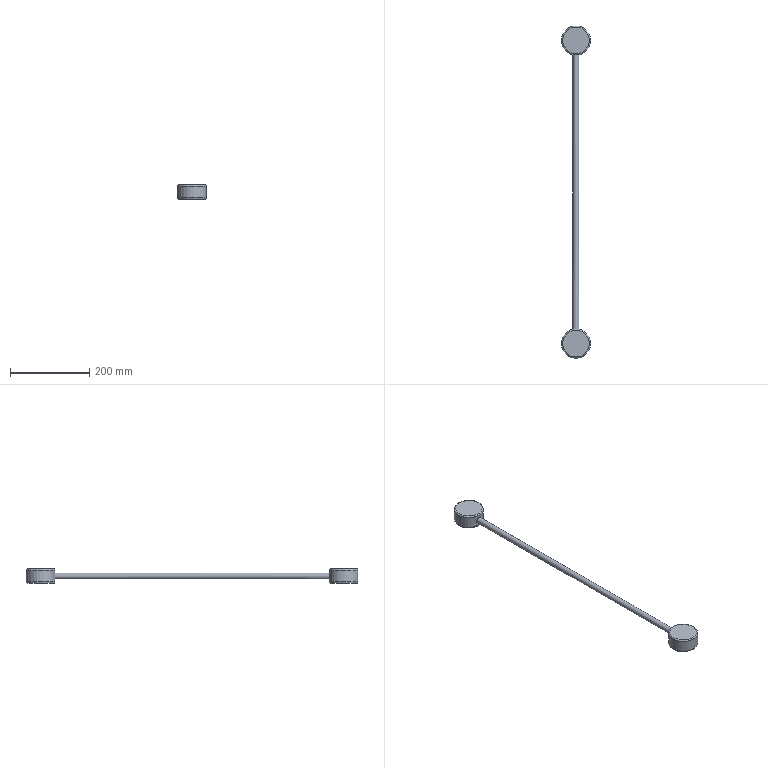Component | NX | LIFTING_ROD | 1 solid | 11 faces | box 73.5 x 839.5 x 36.22 mm | volume 428046 mm3 | plane 4 | torus 4 | cylinder 3 | commonest cylinder face diameters 73.505 x2 15 x1
STEP:
#1=CARTESIAN_POINT('',(0.,0.,0.));
#2=DIRECTION('',(0.,0.,1.));
#3=DIRECTION('',(1.,0.,0.));
#4=AXIS2_PLACEMENT_3D('',#1,#2,#3);
#5=CARTESIAN_POINT('',(33.745,-346.249,-596.264));
#6=VERTEX_POINT('',#5);
#7=CARTESIAN_POINT('',(31.757,-346.262,-596.264));
#8=CARTESIAN_POINT('',(35.732,-346.235,-596.264));
#9=CARTESIAN_POINT('',(37.671,-346.405,-595.446));
#10=CARTESIAN_POINT('',(40.43,-346.788,-592.684));
#11=CARTESIAN_POINT('',(41.244,-346.969,-590.728));
#12=CARTESIAN_POINT('',(41.245,-346.969,-586.803));
#13=CARTESIAN_POINT('',(40.441,-346.789,-584.852));
#14=CARTESIAN_POINT('',(37.65,-346.402,-582.065));
#15=CARTESIAN_POINT('',(35.701,-346.235,-581.263));
#16=CARTESIAN_POINT('',(31.78,-346.263,-581.266));
#17=CARTESIAN_POINT('',(29.825,-346.459,-582.078));
#18=CARTESIAN_POINT('',(27.06,-346.882,-584.842));
#19=CARTESIAN_POINT('',(26.245,-347.075,-586.782));
#20=CARTESIAN_POINT('',(26.244,-347.075,-590.744));
#21=CARTESIAN_POINT('',(27.062,-346.882,-592.687));
#22=CARTESIAN_POINT('',(29.816,-346.46,-595.444));
#23=CARTESIAN_POINT('',(31.757,-346.262,-596.264));
#24=CARTESIAN_POINT('',(35.732,-346.235,-596.264));
#25=B_SPLINE_CURVE_WITH_KNOTS('',3,(#7,#8,#9,#10,#11,#12,#13,#14,#15,#16,#17,#18,#19,#20,#21,#22,#23,#24),.UNSPECIFIED.,.T.,.F.,(2,2,2,2,2,2,2,2,2,2,2),(-0.125,0.,0.125,0.25,0.375,0.5,0.625,0.75,0.875,1.,1.125),.UNSPECIFIED.);
#26=CARTESIAN_POINT('',(33.745,-33.,-588.764));
#27=DIRECTION('',(0.,-1.,0.));
#28=DIRECTION('',(0.,0.,-1.));
#29=AXIS2_PLACEMENT_3D('',#26,#27,#28);
#30=CYLINDRICAL_SURFACE('',#29,7.5);
#31=CARTESIAN_POINT('',(-0.,313.249));
#32=CARTESIAN_POINT('',(0.04815,313.246));
#33=CARTESIAN_POINT('',(0.1441,313.253));
#34=CARTESIAN_POINT('',(0.2874,313.295));
#35=CARTESIAN_POINT('',(0.4303,313.361));
#36=CARTESIAN_POINT('',(0.5728,313.446));
#37=CARTESIAN_POINT('',(0.7149,313.544));
#38=CARTESIAN_POINT('',(0.8568,313.649));
#39=CARTESIAN_POINT('',(0.9992,313.749));
#40=CARTESIAN_POINT('',(1.142,313.838));
#41=CARTESIAN_POINT('',(1.285,313.909));
#42=CARTESIAN_POINT('',(1.428,313.957));
#43=CARTESIAN_POINT('',(1.571,313.975));
#44=CARTESIAN_POINT('',(1.713,313.957));
#45=CARTESIAN_POINT('',(1.856,313.909));
#46=CARTESIAN_POINT('',(1.999,313.838));
#47=CARTESIAN_POINT('',(2.142,313.749));
#48=CARTESIAN_POINT('',(2.285,313.649));
#49=CARTESIAN_POINT('',(2.428,313.542));
#50=CARTESIAN_POINT('',(2.571,313.444));
#51=CARTESIAN_POINT('',(2.714,313.359));
#52=CARTESIAN_POINT('',(2.857,313.294));
#53=CARTESIAN_POINT('',(3.,313.253));
#54=CARTESIAN_POINT('',(3.142,313.243));
#55=CARTESIAN_POINT('',(3.285,313.268));
#56=CARTESIAN_POINT('',(3.428,313.324));
#57=CARTESIAN_POINT('',(3.571,313.404));
#58=CARTESIAN_POINT('',(3.713,313.502));
#59=CARTESIAN_POINT('',(3.856,313.612));
#60=CARTESIAN_POINT('',(3.998,313.729));
#61=CARTESIAN_POINT('',(4.14,313.838));
#62=CARTESIAN_POINT('',(4.283,313.934));
#63=CARTESIAN_POINT('',(4.425,314.011));
#64=CARTESIAN_POINT('',(4.568,314.062));
#65=CARTESIAN_POINT('',(4.712,314.082));
#66=CARTESIAN_POINT('',(4.856,314.063));
#67=CARTESIAN_POINT('',(4.999,314.011));
#68=CARTESIAN_POINT('',(5.142,313.934));
#69=CARTESIAN_POINT('',(5.285,313.838));
#70=CARTESIAN_POINT('',(5.427,313.729));
#71=CARTESIAN_POINT('',(5.568,313.613));
#72=CARTESIAN_POINT('',(5.71,313.503));
#73=CARTESIAN_POINT('',(5.853,313.405));
#74=CARTESIAN_POINT('',(5.996,313.324));
#75=CARTESIAN_POINT('',(6.139,313.268));
#76=CARTESIAN_POINT('',(6.235,313.251));
#77=CARTESIAN_POINT('',(6.283,313.249));
#78=B_SPLINE_CURVE_WITH_KNOTS('',3,(#31,#32,#33,#34,#35,#36,#37,#38,#39,#40,#41,#42,#43,#44,#45,#46,#47,#48,#49,#50,#51,#52,#53,#54,#55,#56,#57,#58,#59,#60,#61,#62,#63,#64,#65,#66,#67,#68,#69,#70,#71,#72,#73,#74,#75,#76,#77),.UNSPECIFIED.,.F.,.F.,(4,1,1,1,1,1,1,1,1,1,1,1,1,1,1,1,1,1,1,1,1,1,1,1,1,1,1,1,1,1,1,1,1,1,1,1,1,1,1,1,1,1,1,1,4),(0.,0.02273,0.04545,0.06818,0.09091,0.1136,0.1364,0.1591,0.1818,0.2045,0.2273,0.25,0.2727,0.2955,0.3182,0.3409,0.3636,0.3864,0.4091,0.4318,0.4545,0.4773,0.5,0.5227,0.5455,0.5682,0.5909,0.6136,0.6364,0.6591,0.6818,0.7045,0.7273,0.75,0.7727,0.7955,0.8182,0.8409,0.8636,0.8864,0.9091,0.9318,0.9545,0.9773,1.),.QUASI_UNIFORM_KNOTS.);
#79=(GEOMETRIC_REPRESENTATION_CONTEXT(2)PARAMETRIC_REPRESENTATION_CONTEXT()REPRESENTATION_CONTEXT('',''));
#80=DEFINITIONAL_REPRESENTATION('',(#78),#79);
#81=PCURVE('',#30,#80);
#82=CARTESIAN_POINT('',(34.,-383.,-570.654));
#83=DIRECTION('',(-0.,0.,-1.));
#84=DIRECTION('',(-1.,0.,0.));
#85=AXIS2_PLACEMENT_3D('',#82,#83,#84);
#86=CYLINDRICAL_SURFACE('',#85,36.752);
#87=CARTESIAN_POINT('',(1.564,25.61));
#88=CARTESIAN_POINT('',(1.574,25.61));
#89=CARTESIAN_POINT('',(1.593,25.556));
#90=CARTESIAN_POINT('',(1.622,25.322));
#91=CARTESIAN_POINT('',(1.649,24.944));
#92=CARTESIAN_POINT('',(1.675,24.431));
#93=CARTESIAN_POINT('',(1.698,23.793));
#94=CARTESIAN_POINT('',(1.719,23.038));
#95=CARTESIAN_POINT('',(1.737,22.178));
#96=CARTESIAN_POINT('',(1.751,21.235));
#97=CARTESIAN_POINT('',(1.761,20.229));
#98=CARTESIAN_POINT('',(1.768,19.181));
#99=CARTESIAN_POINT('',(1.77,18.111));
#100=CARTESIAN_POINT('',(1.768,17.041));
#101=CARTESIAN_POINT('',(1.761,15.994));
#102=CARTESIAN_POINT('',(1.751,14.988));
#103=CARTESIAN_POINT('',(1.737,14.044));
#104=CARTESIAN_POINT('',(1.719,13.181));
#105=CARTESIAN_POINT('',(1.698,12.419));
#106=CARTESIAN_POINT('',(1.675,11.779));
#107=CARTESIAN_POINT('',(1.649,11.268));
#108=CARTESIAN_POINT('',(1.621,10.893));
#109=CARTESIAN_POINT('',(1.593,10.663));
#110=CARTESIAN_POINT('',(1.564,10.583));
#111=CARTESIAN_POINT('',(1.535,10.664));
#112=CARTESIAN_POINT('',(1.506,10.898));
#113=CARTESIAN_POINT('',(1.479,11.274));
#114=CARTESIAN_POINT('',(1.453,11.786));
#115=CARTESIAN_POINT('',(1.429,12.423));
#116=CARTESIAN_POINT('',(1.408,13.179));
#117=CARTESIAN_POINT('',(1.391,14.037));
#118=CARTESIAN_POINT('',(1.377,14.977));
#119=CARTESIAN_POINT('',(1.366,15.981));
#120=CARTESIAN_POINT('',(1.36,17.03));
#121=CARTESIAN_POINT('',(1.357,18.108));
#122=CARTESIAN_POINT('',(1.36,19.187));
#123=CARTESIAN_POINT('',(1.366,20.237));
#124=CARTESIAN_POINT('',(1.377,21.242));
#125=CARTESIAN_POINT('',(1.391,22.182));
#126=CARTESIAN_POINT('',(1.408,23.039));
#127=CARTESIAN_POINT('',(1.429,23.792));
#128=CARTESIAN_POINT('',(1.453,24.43));
#129=CARTESIAN_POINT('',(1.478,24.943));
#130=CARTESIAN_POINT('',(1.506,25.321));
#131=CARTESIAN_POINT('',(1.534,25.556));
#132=CARTESIAN_POINT('',(1.554,25.61));
#133=CARTESIAN_POINT('',(1.564,25.61));
#134=B_SPLINE_CURVE_WITH_KNOTS('',3,(#87,#88,#89,#90,#91,#92,#93,#94,#95,#96,#97,#98,#99,#100,#101,#102,#103,#104,#105,#106,#107,#108,#109,#110,#111,#112,#113,#114,#115,#116,#117,#118,#119,#120,#121,#122,#123,#124,#125,#126,#127,#128,#129,#130,#131,#132,#133),.UNSPECIFIED.,.T.,.F.,(4,1,1,1,1,1,1,1,1,1,1,1,1,1,1,1,1,1,1,1,1,1,1,1,1,1,1,1,1,1,1,1,1,1,1,1,1,1,1,1,1,1,1,1,4),(0.,0.02273,0.04545,0.06818,0.09091,0.1136,0.1364,0.1591,0.1818,0.2045,0.2273,0.25,0.2727,0.2955,0.3182,0.3409,0.3636,0.3864,0.4091,0.4318,0.4545,0.4773,0.5,0.5227,0.5455,0.5682,0.5909,0.6136,0.6364,0.6591,0.6818,0.7045,0.7273,0.75,0.7727,0.7955,0.8182,0.8409,0.8636,0.8864,0.9091,0.9318,0.9545,0.9773,1.),.QUASI_UNIFORM_KNOTS.);
#135=(GEOMETRIC_REPRESENTATION_CONTEXT(2)PARAMETRIC_REPRESENTATION_CONTEXT()REPRESENTATION_CONTEXT('',''));
#136=DEFINITIONAL_REPRESENTATION('',(#134),#135);
#137=PCURVE('',#86,#136);
#138=SURFACE_CURVE('',#25,(#81,#137),.PCURVE_S1.);
#139=EDGE_CURVE('',#6,#6,#138,.T.);
#140=ORIENTED_EDGE('',*,*,#139,.F.);
#141=CARTESIAN_POINT('',(33.745,346.249,-596.264));
#142=VERTEX_POINT('',#141);
#143=CARTESIAN_POINT('',(33.745,346.249,-596.264));
#144=CARTESIAN_POINT('',(33.745,-346.249,-596.264));
#145=B_SPLINE_CURVE_WITH_KNOTS('',1,(#143,#144),.UNSPECIFIED.,.F.,.F.,(2,2),(-379.249,313.249),.PIECEWISE_BEZIER_KNOTS.);
#146=CARTESIAN_POINT('',(-0.,0.));
#147=DIRECTION('',(0.,1.));
#148=VECTOR('',#147,1.);
#149=LINE('',#146,#148);
#150=(GEOMETRIC_REPRESENTATION_CONTEXT(2)PARAMETRIC_REPRESENTATION_CONTEXT()REPRESENTATION_CONTEXT('',''));
#151=DEFINITIONAL_REPRESENTATION('',(#149),#150);
#152=PCURVE('',#30,#151);
#153=CARTESIAN_POINT('',(6.283,0.));
#154=DIRECTION('',(0.,1.));
#155=VECTOR('',#154,1.);
#156=LINE('',#153,#155);
#157=(GEOMETRIC_REPRESENTATION_CONTEXT(2)PARAMETRIC_REPRESENTATION_CONTEXT()REPRESENTATION_CONTEXT('',''));
#158=DEFINITIONAL_REPRESENTATION('',(#156),#157);
#159=PCURVE('',#30,#158);
#160=SEAM_CURVE('',#145,(#152,#159),.PCURVE_S1.);
#161=EDGE_CURVE('',#142,#6,#160,.T.);
#162=ORIENTED_EDGE('',*,*,#161,.F.);
#163=CARTESIAN_POINT('',(35.732,346.235,-596.264));
#164=CARTESIAN_POINT('',(31.757,346.262,-596.264));
#165=CARTESIAN_POINT('',(29.821,346.459,-595.447));
#166=CARTESIAN_POINT('',(27.063,346.881,-592.69));
#167=CARTESIAN_POINT('',(26.247,347.075,-590.735));
#168=CARTESIAN_POINT('',(26.242,347.076,-586.811));
#169=CARTESIAN_POINT('',(27.045,346.884,-584.86));
#170=CARTESIAN_POINT('',(29.829,346.458,-582.071));
#171=CARTESIAN_POINT('',(31.774,346.263,-581.267));
#172=CARTESIAN_POINT('',(35.695,346.235,-581.262));
#173=CARTESIAN_POINT('',(37.654,346.403,-582.072));
#174=CARTESIAN_POINT('',(40.425,346.787,-584.834));
#175=CARTESIAN_POINT('',(41.242,346.968,-586.775));
#176=CARTESIAN_POINT('',(41.247,346.969,-590.737));
#177=CARTESIAN_POINT('',(40.431,346.788,-592.681));
#178=CARTESIAN_POINT('',(37.676,346.406,-595.443));
#179=CARTESIAN_POINT('',(35.732,346.235,-596.264));
#180=CARTESIAN_POINT('',(31.757,346.262,-596.264));
#181=B_SPLINE_CURVE_WITH_KNOTS('',3,(#163,#164,#165,#166,#167,#168,#169,#170,#171,#172,#173,#174,#175,#176,#177,#178,#179,#180),.UNSPECIFIED.,.T.,.F.,(2,2,2,2,2,2,2,2,2,2,2),(-0.125,0.,0.125,0.25,0.375,0.5,0.625,0.75,0.875,1.,1.125),.UNSPECIFIED.);
#182=CARTESIAN_POINT('',(6.283,-379.249));
#183=CARTESIAN_POINT('',(6.235,-379.251));
#184=CARTESIAN_POINT('',(6.139,-379.268));
#185=CARTESIAN_POINT('',(5.996,-379.324));
#186=CARTESIAN_POINT('',(5.853,-379.404));
#187=CARTESIAN_POINT('',(5.711,-379.502));
#188=CARTESIAN_POINT('',(5.569,-379.612));
#189=CARTESIAN_POINT('',(5.427,-379.729));
#190=CARTESIAN_POINT('',(5.285,-379.838));
#191=CARTESIAN_POINT('',(5.142,-379.934));
#192=CARTESIAN_POINT('',(4.999,-380.011));
#193=CARTESIAN_POINT('',(4.856,-380.062));
#194=CARTESIAN_POINT('',(4.713,-380.082));
#195=CARTESIAN_POINT('',(4.571,-380.063));
#196=CARTESIAN_POINT('',(4.428,-380.012));
#197=CARTESIAN_POINT('',(4.285,-379.936));
#198=CARTESIAN_POINT('',(4.142,-379.84));
#199=CARTESIAN_POINT('',(4.,-379.73));
#200=CARTESIAN_POINT('',(3.856,-379.612));
#201=CARTESIAN_POINT('',(3.713,-379.502));
#202=CARTESIAN_POINT('',(3.571,-379.404));
#203=CARTESIAN_POINT('',(3.428,-379.324));
#204=CARTESIAN_POINT('',(3.285,-379.268));
#205=CARTESIAN_POINT('',(3.143,-379.243));
#206=CARTESIAN_POINT('',(3.,-379.253));
#207=CARTESIAN_POINT('',(2.857,-379.294));
#208=CARTESIAN_POINT('',(2.714,-379.36));
#209=CARTESIAN_POINT('',(2.571,-379.444));
#210=CARTESIAN_POINT('',(2.429,-379.542));
#211=CARTESIAN_POINT('',(2.287,-379.648));
#212=CARTESIAN_POINT('',(2.144,-379.748));
#213=CARTESIAN_POINT('',(2.002,-379.837));
#214=CARTESIAN_POINT('',(1.859,-379.909));
#215=CARTESIAN_POINT('',(1.716,-379.957));
#216=CARTESIAN_POINT('',(1.572,-379.975));
#217=CARTESIAN_POINT('',(1.428,-379.957));
#218=CARTESIAN_POINT('',(1.285,-379.909));
#219=CARTESIAN_POINT('',(1.142,-379.838));
#220=CARTESIAN_POINT('',(0.9995,-379.749));
#221=CARTESIAN_POINT('',(0.8573,-379.65));
#222=CARTESIAN_POINT('',(0.7156,-379.544));
#223=CARTESIAN_POINT('',(0.5734,-379.446));
#224=CARTESIAN_POINT('',(0.4307,-379.361));
#225=CARTESIAN_POINT('',(0.2876,-379.295));
#226=CARTESIAN_POINT('',(0.1442,-379.253));
#227=CARTESIAN_POINT('',(0.04815,-379.246));
#228=CARTESIAN_POINT('',(-0.,-379.249));
#229=B_SPLINE_CURVE_WITH_KNOTS('',3,(#182,#183,#184,#185,#186,#187,#188,#189,#190,#191,#192,#193,#194,#195,#196,#197,#198,#199,#200,#201,#202,#203,#204,#205,#206,#207,#208,#209,#210,#211,#212,#213,#214,#215,#216,#217,#218,#219,#220,#221,#222,#223,#224,#225,#226,#227,#228),.UNSPECIFIED.,.F.,.F.,(4,1,1,1,1,1,1,1,1,1,1,1,1,1,1,1,1,1,1,1,1,1,1,1,1,1,1,1,1,1,1,1,1,1,1,1,1,1,1,1,1,1,1,1,4),(0.,0.02273,0.04545,0.06818,0.09091,0.1136,0.1364,0.1591,0.1818,0.2045,0.2273,0.25,0.2727,0.2955,0.3182,0.3409,0.3636,0.3864,0.4091,0.4318,0.4545,0.4773,0.5,0.5227,0.5455,0.5682,0.5909,0.6136,0.6364,0.6591,0.6818,0.7045,0.7273,0.75,0.7727,0.7955,0.8182,0.8409,0.8636,0.8864,0.9091,0.9318,0.9545,0.9773,1.),.QUASI_UNIFORM_KNOTS.);
#230=(GEOMETRIC_REPRESENTATION_CONTEXT(2)PARAMETRIC_REPRESENTATION_CONTEXT()REPRESENTATION_CONTEXT('',''));
#231=DEFINITIONAL_REPRESENTATION('',(#229),#230);
#232=PCURVE('',#30,#231);
#233=CARTESIAN_POINT('',(34.,383.,-570.654));
#234=DIRECTION('',(-0.,0.,-1.));
#235=DIRECTION('',(-1.,0.,0.));
#236=AXIS2_PLACEMENT_3D('',#233,#234,#235);
#237=CYLINDRICAL_SURFACE('',#236,36.752);
#238=CARTESIAN_POINT('',(4.719,25.61));
#239=CARTESIAN_POINT('',(4.729,25.61));
#240=CARTESIAN_POINT('',(4.749,25.556));
#241=CARTESIAN_POINT('',(4.777,25.322));
#242=CARTESIAN_POINT('',(4.805,24.945));
#243=CARTESIAN_POINT('',(4.83,24.433));
#244=CARTESIAN_POINT('',(4.854,23.796));
#245=CARTESIAN_POINT('',(4.875,23.042));
#246=CARTESIAN_POINT('',(4.892,22.183));
#247=CARTESIAN_POINT('',(4.906,21.241));
#248=CARTESIAN_POINT('',(4.917,20.236));
#249=CARTESIAN_POINT('',(4.923,19.188));
#250=CARTESIAN_POINT('',(4.926,18.118));
#251=CARTESIAN_POINT('',(4.924,17.049));
#252=CARTESIAN_POINT('',(4.917,16.002));
#253=CARTESIAN_POINT('',(4.907,14.996));
#254=CARTESIAN_POINT('',(4.893,14.052));
#255=CARTESIAN_POINT('',(4.875,13.188));
#256=CARTESIAN_POINT('',(4.854,12.426));
#257=CARTESIAN_POINT('',(4.83,11.785));
#258=CARTESIAN_POINT('',(4.805,11.273));
#259=CARTESIAN_POINT('',(4.777,10.897));
#260=CARTESIAN_POINT('',(4.749,10.665));
#261=CARTESIAN_POINT('',(4.72,10.583));
#262=CARTESIAN_POINT('',(4.691,10.662));
#263=CARTESIAN_POINT('',(4.662,10.894));
#264=CARTESIAN_POINT('',(4.635,11.269));
#265=CARTESIAN_POINT('',(4.609,11.78));
#266=CARTESIAN_POINT('',(4.585,12.416));
#267=CARTESIAN_POINT('',(4.564,13.172));
#268=CARTESIAN_POINT('',(4.547,14.029));
#269=CARTESIAN_POINT('',(4.533,14.969));
#270=CARTESIAN_POINT('',(4.522,15.974));
#271=CARTESIAN_POINT('',(4.516,17.023));
#272=CARTESIAN_POINT('',(4.513,18.101));
#273=CARTESIAN_POINT('',(4.515,19.18));
#274=CARTESIAN_POINT('',(4.522,20.23));
#275=CARTESIAN_POINT('',(4.532,21.236));
#276=CARTESIAN_POINT('',(4.546,22.177));
#277=CARTESIAN_POINT('',(4.564,23.035));
#278=CARTESIAN_POINT('',(4.585,23.79));
#279=CARTESIAN_POINT('',(4.608,24.428));
#280=CARTESIAN_POINT('',(4.634,24.942));
#281=CARTESIAN_POINT('',(4.661,25.321));
#282=CARTESIAN_POINT('',(4.69,25.556));
#283=CARTESIAN_POINT('',(4.71,25.61));
#284=CARTESIAN_POINT('',(4.719,25.61));
#285=B_SPLINE_CURVE_WITH_KNOTS('',3,(#238,#239,#240,#241,#242,#243,#244,#245,#246,#247,#248,#249,#250,#251,#252,#253,#254,#255,#256,#257,#258,#259,#260,#261,#262,#263,#264,#265,#266,#267,#268,#269,#270,#271,#272,#273,#274,#275,#276,#277,#278,#279,#280,#281,#282,#283,#284),.UNSPECIFIED.,.T.,.F.,(4,1,1,1,1,1,1,1,1,1,1,1,1,1,1,1,1,1,1,1,1,1,1,1,1,1,1,1,1,1,1,1,1,1,1,1,1,1,1,1,1,1,1,1,4),(0.,0.02273,0.04545,0.06818,0.09091,0.1136,0.1364,0.1591,0.1818,0.2045,0.2273,0.25,0.2727,0.2955,0.3182,0.3409,0.3636,0.3864,0.4091,0.4318,0.4545,0.4773,0.5,0.5227,0.5455,0.5682,0.5909,0.6136,0.6364,0.6591,0.6818,0.7045,0.7273,0.75,0.7727,0.7955,0.8182,0.8409,0.8636,0.8864,0.9091,0.9318,0.9545,0.9773,1.),.QUASI_UNIFORM_KNOTS.);
#286=(GEOMETRIC_REPRESENTATION_CONTEXT(2)PARAMETRIC_REPRESENTATION_CONTEXT()REPRESENTATION_CONTEXT('',''));
#287=DEFINITIONAL_REPRESENTATION('',(#285),#286);
#288=PCURVE('',#237,#287);
#289=SURFACE_CURVE('',#181,(#232,#288),.PCURVE_S1.);
#290=EDGE_CURVE('',#142,#142,#289,.T.);
#291=ORIENTED_EDGE('',*,*,#290,.F.);
#292=ORIENTED_EDGE('',*,*,#161,.T.);
#293=EDGE_LOOP('',(#140,#162,#291,#292));
#294=FACE_BOUND('',#293,.T.);
#295=ADVANCED_FACE('',(#294),#30,.T.);
#296=CARTESIAN_POINT('',(-2.752,-383.,-573.654));
#297=VERTEX_POINT('',#296);
#298=CARTESIAN_POINT('',(34.,-383.,-573.654));
#299=DIRECTION('',(-0.,0.,-1.));
#300=DIRECTION('',(-1.,0.,0.));
#301=AXIS2_PLACEMENT_3D('',#298,#299,#300);
#302=CIRCLE('',#301,36.752);
#303=CARTESIAN_POINT('',(0.,3.));
#304=DIRECTION('',(1.,0.));
#305=VECTOR('',#304,1.);
#306=LINE('',#303,#305);
#307=(GEOMETRIC_REPRESENTATION_CONTEXT(2)PARAMETRIC_REPRESENTATION_CONTEXT()REPRESENTATION_CONTEXT('',''));
#308=DEFINITIONAL_REPRESENTATION('',(#306),#307);
#309=PCURVE('',#86,#308);
#310=CARTESIAN_POINT('',(34.,-383.,-573.654));
#311=DIRECTION('',(-0.,0.,-1.));
#312=DIRECTION('',(-1.,0.,0.));
#313=AXIS2_PLACEMENT_3D('',#310,#311,#312);
#314=TOROIDAL_SURFACE('',#313,33.752,3.);
#315=CARTESIAN_POINT('',(0.,6.283));
#316=DIRECTION('',(1.,0.));
#317=VECTOR('',#316,1.);
#318=LINE('',#315,#317);
#319=(GEOMETRIC_REPRESENTATION_CONTEXT(2)PARAMETRIC_REPRESENTATION_CONTEXT()REPRESENTATION_CONTEXT('',''));
#320=DEFINITIONAL_REPRESENTATION('',(#318),#319);
#321=PCURVE('',#314,#320);
#322=SURFACE_CURVE('',#302,(#309,#321),.PCURVE_S1.);
#323=EDGE_CURVE('',#297,#297,#322,.T.);
#324=ORIENTED_EDGE('',*,*,#323,.T.);
#325=CARTESIAN_POINT('',(-2.752,-383.,-603.874));
#326=VERTEX_POINT('',#325);
#327=CARTESIAN_POINT('',(-2.752,-383.,-573.654));
#328=CARTESIAN_POINT('',(-2.752,-383.,-603.874));
#329=B_SPLINE_CURVE_WITH_KNOTS('',1,(#327,#328),.UNSPECIFIED.,.F.,.F.,(2,2),(3.,33.22),.PIECEWISE_BEZIER_KNOTS.);
#330=CARTESIAN_POINT('',(6.283,0.));
#331=DIRECTION('',(0.,1.));
#332=VECTOR('',#331,1.);
#333=LINE('',#330,#332);
#334=(GEOMETRIC_REPRESENTATION_CONTEXT(2)PARAMETRIC_REPRESENTATION_CONTEXT()REPRESENTATION_CONTEXT('',''));
#335=DEFINITIONAL_REPRESENTATION('',(#333),#334);
#336=PCURVE('',#86,#335);
#337=CARTESIAN_POINT('',(0.,0.));
#338=DIRECTION('',(0.,1.));
#339=VECTOR('',#338,1.);
#340=LINE('',#337,#339);
#341=(GEOMETRIC_REPRESENTATION_CONTEXT(2)PARAMETRIC_REPRESENTATION_CONTEXT()REPRESENTATION_CONTEXT('',''));
#342=DEFINITIONAL_REPRESENTATION('',(#340),#341);
#343=PCURVE('',#86,#342);
#344=SEAM_CURVE('',#329,(#336,#343),.PCURVE_S1.);
#345=EDGE_CURVE('',#297,#326,#344,.T.);
#346=ORIENTED_EDGE('',*,*,#345,.T.);
#347=CARTESIAN_POINT('',(34.,-383.,-603.874));
#348=DIRECTION('',(0.,0.,1.));
#349=DIRECTION('',(-1.,0.,0.));
#350=AXIS2_PLACEMENT_3D('',#347,#348,#349);
#351=CIRCLE('',#350,36.752);
#352=CARTESIAN_POINT('',(6.283,33.22));
#353=DIRECTION('',(-1.,0.));
#354=VECTOR('',#353,1.);
#355=LINE('',#352,#354);
#356=(GEOMETRIC_REPRESENTATION_CONTEXT(2)PARAMETRIC_REPRESENTATION_CONTEXT()REPRESENTATION_CONTEXT('',''));
#357=DEFINITIONAL_REPRESENTATION('',(#355),#356);
#358=PCURVE('',#86,#357);
#359=CARTESIAN_POINT('',(34.,-383.,-603.874));
#360=DIRECTION('',(-0.,0.,-1.));
#361=DIRECTION('',(-1.,0.,0.));
#362=AXIS2_PLACEMENT_3D('',#359,#360,#361);
#363=TOROIDAL_SURFACE('',#362,33.752,3.);
#364=CARTESIAN_POINT('',(6.283,6.283));
#365=DIRECTION('',(-1.,0.));
#366=VECTOR('',#365,1.);
#367=LINE('',#364,#366);
#368=(GEOMETRIC_REPRESENTATION_CONTEXT(2)PARAMETRIC_REPRESENTATION_CONTEXT()REPRESENTATION_CONTEXT('',''));
#369=DEFINITIONAL_REPRESENTATION('',(#367),#368);
#370=PCURVE('',#363,#369);
#371=SURFACE_CURVE('',#351,(#358,#370),.PCURVE_S1.);
#372=EDGE_CURVE('',#326,#326,#371,.T.);
#373=ORIENTED_EDGE('',*,*,#372,.T.);
#374=ORIENTED_EDGE('',*,*,#345,.F.);
#375=EDGE_LOOP('',(#324,#346,#373,#374));
#376=FACE_BOUND('',#375,.T.);
#377=ORIENTED_EDGE('',*,*,#139,.T.);
#378=EDGE_LOOP('',(#377));
#379=FACE_BOUND('',#378,.T.);
#380=ADVANCED_FACE('',(#376,#379),#86,.T.);
#381=CARTESIAN_POINT('',(0.2477,-383.,-570.654));
#382=VERTEX_POINT('',#381);
#383=CARTESIAN_POINT('',(34.,-383.,-570.654));
#384=DIRECTION('',(0.,0.,1.));
#385=DIRECTION('',(-1.,0.,0.));
#386=AXIS2_PLACEMENT_3D('',#383,#384,#385);
#387=CIRCLE('',#386,33.752);
#388=CARTESIAN_POINT('',(34.,-383.,-570.654));
#389=DIRECTION('',(-0.,0.,-1.));
#390=DIRECTION('',(-1.,0.,0.));
#391=AXIS2_PLACEMENT_3D('',#388,#389,#390);
#392=PLANE('',#391);
#393=CARTESIAN_POINT('',(33.752,0.));
#394=CARTESIAN_POINT('',(33.752,-58.461));
#395=CARTESIAN_POINT('',(-16.876,-29.23));
#396=CARTESIAN_POINT('',(-67.505,-0.));
#397=CARTESIAN_POINT('',(-16.876,29.23));
#398=CARTESIAN_POINT('',(33.752,58.461));
#399=CARTESIAN_POINT('',(33.752,0.));
#400=(BOUNDED_CURVE()B_SPLINE_CURVE(2,(#393,#394,#395,#396,#397,#398,#399),.UNSPECIFIED.,.T.,.F.)B_SPLINE_CURVE_WITH_KNOTS((1,2,2,2,2,1),(-2.094,0.,2.094,4.189,6.283,8.378),.UNSPECIFIED.)CURVE()GEOMETRIC_REPRESENTATION_ITEM()RATIONAL_B_SPLINE_CURVE((1.,0.5,1.,0.5,1.,0.5,1.))REPRESENTATION_ITEM(''));
#401=(GEOMETRIC_REPRESENTATION_CONTEXT(2)PARAMETRIC_REPRESENTATION_CONTEXT()REPRESENTATION_CONTEXT('',''));
#402=DEFINITIONAL_REPRESENTATION('',(#400),#401);
#403=PCURVE('',#392,#402);
#404=CARTESIAN_POINT('',(6.283,4.712));
#405=DIRECTION('',(-1.,0.));
#406=VECTOR('',#405,1.);
#407=LINE('',#404,#406);
#408=(GEOMETRIC_REPRESENTATION_CONTEXT(2)PARAMETRIC_REPRESENTATION_CONTEXT()REPRESENTATION_CONTEXT('',''));
#409=DEFINITIONAL_REPRESENTATION('',(#407),#408);
#410=PCURVE('',#314,#409);
#411=SURFACE_CURVE('',#387,(#403,#410),.PCURVE_S1.);
#412=EDGE_CURVE('',#382,#382,#411,.T.);
#413=ORIENTED_EDGE('',*,*,#412,.T.);
#414=EDGE_LOOP('',(#413));
#415=FACE_BOUND('',#414,.T.);
#416=ADVANCED_FACE('',(#415),#392,.F.);
#417=CARTESIAN_POINT('',(0.2477,-383.,-606.874));
#418=VERTEX_POINT('',#417);
#419=CARTESIAN_POINT('',(34.,-383.,-606.874));
#420=DIRECTION('',(-0.,0.,-1.));
#421=DIRECTION('',(-1.,0.,0.));
#422=AXIS2_PLACEMENT_3D('',#419,#420,#421);
#423=CIRCLE('',#422,33.752);
#424=CARTESIAN_POINT('',(34.,-383.,-606.874));
#425=DIRECTION('',(-0.,0.,-1.));
#426=DIRECTION('',(-1.,0.,0.));
#427=AXIS2_PLACEMENT_3D('',#424,#425,#426);
#428=PLANE('',#427);
#429=CARTESIAN_POINT('',(0.,0.));
#430=DIRECTION('',(1.,0.));
#431=AXIS2_PLACEMENT_2D('',#429,#430);
#432=CIRCLE('',#431,33.752);
#433=(GEOMETRIC_REPRESENTATION_CONTEXT(2)PARAMETRIC_REPRESENTATION_CONTEXT()REPRESENTATION_CONTEXT('',''));
#434=DEFINITIONAL_REPRESENTATION('',(#432),#433);
#435=PCURVE('',#428,#434);
#436=CARTESIAN_POINT('',(0.,7.854));
#437=DIRECTION('',(1.,0.));
#438=VECTOR('',#437,1.);
#439=LINE('',#436,#438);
#440=(GEOMETRIC_REPRESENTATION_CONTEXT(2)PARAMETRIC_REPRESENTATION_CONTEXT()REPRESENTATION_CONTEXT('',''));
#441=DEFINITIONAL_REPRESENTATION('',(#439),#440);
#442=PCURVE('',#363,#441);
#443=SURFACE_CURVE('',#423,(#435,#442),.PCURVE_S1.);
#444=EDGE_CURVE('',#418,#418,#443,.T.);
#445=ORIENTED_EDGE('',*,*,#444,.T.);
#446=EDGE_LOOP('',(#445));
#447=FACE_BOUND('',#446,.T.);
#448=ADVANCED_FACE('',(#447),#428,.T.);
#449=ORIENTED_EDGE('',*,*,#372,.F.);
#450=CARTESIAN_POINT('',(-2.752,-383.,-603.874));
#451=CARTESIAN_POINT('',(-2.752,-383.,-604.676));
#452=CARTESIAN_POINT('',(-2.497,-383.,-605.458));
#453=CARTESIAN_POINT('',(-2.008,-383.,-606.13));
#454=CARTESIAN_POINT('',(-1.335,-383.,-606.619));
#455=CARTESIAN_POINT('',(-0.5543,-383.,-606.874));
#456=CARTESIAN_POINT('',(0.2477,-383.,-606.874));
#457=(BOUNDED_CURVE()B_SPLINE_CURVE(6,(#450,#451,#452,#453,#454,#455,#456),.UNSPECIFIED.,.F.,.F.)B_SPLINE_CURVE_WITH_KNOTS((7,7),(0.,1.571),.PIECEWISE_BEZIER_KNOTS.)CURVE()GEOMETRIC_REPRESENTATION_ITEM()RATIONAL_B_SPLINE_CURVE((1.031,1.01,0.9979,0.994,0.9979,1.01,1.031))REPRESENTATION_ITEM(''));
#458=CARTESIAN_POINT('',(6.283,6.283));
#459=DIRECTION('',(0.,1.));
#460=VECTOR('',#459,1.);
#461=LINE('',#458,#460);
#462=(GEOMETRIC_REPRESENTATION_CONTEXT(2)PARAMETRIC_REPRESENTATION_CONTEXT()REPRESENTATION_CONTEXT('',''));
#463=DEFINITIONAL_REPRESENTATION('',(#461),#462);
#464=PCURVE('',#363,#463);
#465=CARTESIAN_POINT('',(0.,6.283));
#466=DIRECTION('',(0.,1.));
#467=VECTOR('',#466,1.);
#468=LINE('',#465,#467);
#469=(GEOMETRIC_REPRESENTATION_CONTEXT(2)PARAMETRIC_REPRESENTATION_CONTEXT()REPRESENTATION_CONTEXT('',''));
#470=DEFINITIONAL_REPRESENTATION('',(#468),#469);
#471=PCURVE('',#363,#470);
#472=SEAM_CURVE('',#457,(#464,#471),.PCURVE_S1.);
#473=EDGE_CURVE('',#326,#418,#472,.T.);
#474=ORIENTED_EDGE('',*,*,#473,.T.);
#475=ORIENTED_EDGE('',*,*,#444,.F.);
#476=ORIENTED_EDGE('',*,*,#473,.F.);
#477=EDGE_LOOP('',(#449,#474,#475,#476));
#478=FACE_BOUND('',#477,.T.);
#479=ADVANCED_FACE('',(#478),#363,.T.);
#480=ORIENTED_EDGE('',*,*,#412,.F.);
#481=CARTESIAN_POINT('',(0.2477,-383.,-570.654));
#482=CARTESIAN_POINT('',(-0.5543,-383.,-570.654));
#483=CARTESIAN_POINT('',(-1.335,-383.,-570.909));
#484=CARTESIAN_POINT('',(-2.008,-383.,-571.399));
#485=CARTESIAN_POINT('',(-2.497,-383.,-572.071));
#486=CARTESIAN_POINT('',(-2.752,-383.,-572.852));
#487=CARTESIAN_POINT('',(-2.752,-383.,-573.654));
#488=(BOUNDED_CURVE()B_SPLINE_CURVE(6,(#481,#482,#483,#484,#485,#486,#487),.UNSPECIFIED.,.F.,.F.)B_SPLINE_CURVE_WITH_KNOTS((7,7),(4.712,6.283),.PIECEWISE_BEZIER_KNOTS.)CURVE()GEOMETRIC_REPRESENTATION_ITEM()RATIONAL_B_SPLINE_CURVE((1.031,1.01,0.9979,0.994,0.9979,1.01,1.031))REPRESENTATION_ITEM(''));
#489=CARTESIAN_POINT('',(6.283,0.));
#490=DIRECTION('',(0.,1.));
#491=VECTOR('',#490,1.);
#492=LINE('',#489,#491);
#493=(GEOMETRIC_REPRESENTATION_CONTEXT(2)PARAMETRIC_REPRESENTATION_CONTEXT()REPRESENTATION_CONTEXT('',''));
#494=DEFINITIONAL_REPRESENTATION('',(#492),#493);
#495=PCURVE('',#314,#494);
#496=CARTESIAN_POINT('',(0.,0.));
#497=DIRECTION('',(0.,1.));
#498=VECTOR('',#497,1.);
#499=LINE('',#496,#498);
#500=(GEOMETRIC_REPRESENTATION_CONTEXT(2)PARAMETRIC_REPRESENTATION_CONTEXT()REPRESENTATION_CONTEXT('',''));
#501=DEFINITIONAL_REPRESENTATION('',(#499),#500);
#502=PCURVE('',#314,#501);
#503=SEAM_CURVE('',#488,(#495,#502),.PCURVE_S1.);
#504=EDGE_CURVE('',#382,#297,#503,.T.);
#505=ORIENTED_EDGE('',*,*,#504,.T.);
#506=ORIENTED_EDGE('',*,*,#323,.F.);
#507=ORIENTED_EDGE('',*,*,#504,.F.);
#508=EDGE_LOOP('',(#480,#505,#506,#507));
#509=FACE_BOUND('',#508,.T.);
#510=ADVANCED_FACE('',(#509),#314,.T.);
#511=CARTESIAN_POINT('',(-2.752,383.,-573.654));
#512=VERTEX_POINT('',#511);
#513=CARTESIAN_POINT('',(34.,383.,-573.654));
#514=DIRECTION('',(-0.,0.,-1.));
#515=DIRECTION('',(-1.,0.,0.));
#516=AXIS2_PLACEMENT_3D('',#513,#514,#515);
#517=CIRCLE('',#516,36.752);
#518=CARTESIAN_POINT('',(0.,3.));
#519=DIRECTION('',(1.,0.));
#520=VECTOR('',#519,1.);
#521=LINE('',#518,#520);
#522=(GEOMETRIC_REPRESENTATION_CONTEXT(2)PARAMETRIC_REPRESENTATION_CONTEXT()REPRESENTATION_CONTEXT('',''));
#523=DEFINITIONAL_REPRESENTATION('',(#521),#522);
#524=PCURVE('',#237,#523);
#525=CARTESIAN_POINT('',(34.,383.,-573.654));
#526=DIRECTION('',(-0.,0.,-1.));
#527=DIRECTION('',(-1.,0.,0.));
#528=AXIS2_PLACEMENT_3D('',#525,#526,#527);
#529=TOROIDAL_SURFACE('',#528,33.752,3.);
#530=CARTESIAN_POINT('',(0.,6.283));
#531=DIRECTION('',(1.,0.));
#532=VECTOR('',#531,1.);
#533=LINE('',#530,#532);
#534=(GEOMETRIC_REPRESENTATION_CONTEXT(2)PARAMETRIC_REPRESENTATION_CONTEXT()REPRESENTATION_CONTEXT('',''));
#535=DEFINITIONAL_REPRESENTATION('',(#533),#534);
#536=PCURVE('',#529,#535);
#537=SURFACE_CURVE('',#517,(#524,#536),.PCURVE_S1.);
#538=EDGE_CURVE('',#512,#512,#537,.T.);
#539=ORIENTED_EDGE('',*,*,#538,.T.);
#540=CARTESIAN_POINT('',(-2.752,383.,-603.874));
#541=VERTEX_POINT('',#540);
#542=CARTESIAN_POINT('',(-2.752,383.,-573.654));
#543=CARTESIAN_POINT('',(-2.752,383.,-603.874));
#544=B_SPLINE_CURVE_WITH_KNOTS('',1,(#542,#543),.UNSPECIFIED.,.F.,.F.,(2,2),(3.,33.22),.PIECEWISE_BEZIER_KNOTS.);
#545=CARTESIAN_POINT('',(6.283,0.));
#546=DIRECTION('',(0.,1.));
#547=VECTOR('',#546,1.);
#548=LINE('',#545,#547);
#549=(GEOMETRIC_REPRESENTATION_CONTEXT(2)PARAMETRIC_REPRESENTATION_CONTEXT()REPRESENTATION_CONTEXT('',''));
#550=DEFINITIONAL_REPRESENTATION('',(#548),#549);
#551=PCURVE('',#237,#550);
#552=CARTESIAN_POINT('',(0.,0.));
#553=DIRECTION('',(0.,1.));
#554=VECTOR('',#553,1.);
#555=LINE('',#552,#554);
#556=(GEOMETRIC_REPRESENTATION_CONTEXT(2)PARAMETRIC_REPRESENTATION_CONTEXT()REPRESENTATION_CONTEXT('',''));
#557=DEFINITIONAL_REPRESENTATION('',(#555),#556);
#558=PCURVE('',#237,#557);
#559=SEAM_CURVE('',#544,(#551,#558),.PCURVE_S1.);
#560=EDGE_CURVE('',#512,#541,#559,.T.);
#561=ORIENTED_EDGE('',*,*,#560,.T.);
#562=CARTESIAN_POINT('',(34.,383.,-603.874));
#563=DIRECTION('',(0.,0.,1.));
#564=DIRECTION('',(-1.,0.,0.));
#565=AXIS2_PLACEMENT_3D('',#562,#563,#564);
#566=CIRCLE('',#565,36.752);
#567=CARTESIAN_POINT('',(6.283,33.22));
#568=DIRECTION('',(-1.,0.));
#569=VECTOR('',#568,1.);
#570=LINE('',#567,#569);
#571=(GEOMETRIC_REPRESENTATION_CONTEXT(2)PARAMETRIC_REPRESENTATION_CONTEXT()REPRESENTATION_CONTEXT('',''));
#572=DEFINITIONAL_REPRESENTATION('',(#570),#571);
#573=PCURVE('',#237,#572);
#574=CARTESIAN_POINT('',(34.,383.,-603.874));
#575=DIRECTION('',(-0.,0.,-1.));
#576=DIRECTION('',(-1.,0.,0.));
#577=AXIS2_PLACEMENT_3D('',#574,#575,#576);
#578=TOROIDAL_SURFACE('',#577,33.752,3.);
#579=CARTESIAN_POINT('',(6.283,6.283));
#580=DIRECTION('',(-1.,0.));
#581=VECTOR('',#580,1.);
#582=LINE('',#579,#581);
#583=(GEOMETRIC_REPRESENTATION_CONTEXT(2)PARAMETRIC_REPRESENTATION_CONTEXT()REPRESENTATION_CONTEXT('',''));
#584=DEFINITIONAL_REPRESENTATION('',(#582),#583);
#585=PCURVE('',#578,#584);
#586=SURFACE_CURVE('',#566,(#573,#585),.PCURVE_S1.);
#587=EDGE_CURVE('',#541,#541,#586,.T.);
#588=ORIENTED_EDGE('',*,*,#587,.T.);
#589=ORIENTED_EDGE('',*,*,#560,.F.);
#590=EDGE_LOOP('',(#539,#561,#588,#589));
#591=FACE_BOUND('',#590,.T.);
#592=ORIENTED_EDGE('',*,*,#290,.T.);
#593=EDGE_LOOP('',(#592));
#594=FACE_BOUND('',#593,.T.);
#595=ADVANCED_FACE('',(#591,#594),#237,.T.);
#596=CARTESIAN_POINT('',(0.2477,383.,-570.654));
#597=VERTEX_POINT('',#596);
#598=CARTESIAN_POINT('',(34.,383.,-570.654));
#599=DIRECTION('',(0.,0.,1.));
#600=DIRECTION('',(-1.,0.,0.));
#601=AXIS2_PLACEMENT_3D('',#598,#599,#600);
#602=CIRCLE('',#601,33.752);
#603=CARTESIAN_POINT('',(34.,383.,-570.654));
#604=DIRECTION('',(-0.,0.,-1.));
#605=DIRECTION('',(-1.,0.,0.));
#606=AXIS2_PLACEMENT_3D('',#603,#604,#605);
#607=PLANE('',#606);
#608=CARTESIAN_POINT('',(33.752,0.));
#609=CARTESIAN_POINT('',(33.752,-58.461));
#610=CARTESIAN_POINT('',(-16.876,-29.23));
#611=CARTESIAN_POINT('',(-67.505,-0.));
#612=CARTESIAN_POINT('',(-16.876,29.23));
#613=CARTESIAN_POINT('',(33.752,58.461));
#614=CARTESIAN_POINT('',(33.752,0.));
#615=(BOUNDED_CURVE()B_SPLINE_CURVE(2,(#608,#609,#610,#611,#612,#613,#614),.UNSPECIFIED.,.T.,.F.)B_SPLINE_CURVE_WITH_KNOTS((1,2,2,2,2,1),(-2.094,0.,2.094,4.189,6.283,8.378),.UNSPECIFIED.)CURVE()GEOMETRIC_REPRESENTATION_ITEM()RATIONAL_B_SPLINE_CURVE((1.,0.5,1.,0.5,1.,0.5,1.))REPRESENTATION_ITEM(''));
#616=(GEOMETRIC_REPRESENTATION_CONTEXT(2)PARAMETRIC_REPRESENTATION_CONTEXT()REPRESENTATION_CONTEXT('',''));
#617=DEFINITIONAL_REPRESENTATION('',(#615),#616);
#618=PCURVE('',#607,#617);
#619=CARTESIAN_POINT('',(6.283,4.712));
#620=DIRECTION('',(-1.,0.));
#621=VECTOR('',#620,1.);
#622=LINE('',#619,#621);
#623=(GEOMETRIC_REPRESENTATION_CONTEXT(2)PARAMETRIC_REPRESENTATION_CONTEXT()REPRESENTATION_CONTEXT('',''));
#624=DEFINITIONAL_REPRESENTATION('',(#622),#623);
#625=PCURVE('',#529,#624);
#626=SURFACE_CURVE('',#602,(#618,#625),.PCURVE_S1.);
#627=EDGE_CURVE('',#597,#597,#626,.T.);
#628=ORIENTED_EDGE('',*,*,#627,.T.);
#629=EDGE_LOOP('',(#628));
#630=FACE_BOUND('',#629,.T.);
#631=ADVANCED_FACE('',(#630),#607,.F.);
#632=CARTESIAN_POINT('',(0.2477,383.,-606.874));
#633=VERTEX_POINT('',#632);
#634=CARTESIAN_POINT('',(34.,383.,-606.874));
#635=DIRECTION('',(-0.,0.,-1.));
#636=DIRECTION('',(-1.,0.,0.));
#637=AXIS2_PLACEMENT_3D('',#634,#635,#636);
#638=CIRCLE('',#637,33.752);
#639=CARTESIAN_POINT('',(34.,383.,-606.874));
#640=DIRECTION('',(-0.,0.,-1.));
#641=DIRECTION('',(-1.,0.,0.));
#642=AXIS2_PLACEMENT_3D('',#639,#640,#641);
#643=PLANE('',#642);
#644=CARTESIAN_POINT('',(0.,0.));
#645=DIRECTION('',(1.,0.));
#646=AXIS2_PLACEMENT_2D('',#644,#645);
#647=CIRCLE('',#646,33.752);
#648=(GEOMETRIC_REPRESENTATION_CONTEXT(2)PARAMETRIC_REPRESENTATION_CONTEXT()REPRESENTATION_CONTEXT('',''));
#649=DEFINITIONAL_REPRESENTATION('',(#647),#648);
#650=PCURVE('',#643,#649);
#651=CARTESIAN_POINT('',(0.,7.854));
#652=DIRECTION('',(1.,0.));
#653=VECTOR('',#652,1.);
#654=LINE('',#651,#653);
#655=(GEOMETRIC_REPRESENTATION_CONTEXT(2)PARAMETRIC_REPRESENTATION_CONTEXT()REPRESENTATION_CONTEXT('',''));
#656=DEFINITIONAL_REPRESENTATION('',(#654),#655);
#657=PCURVE('',#578,#656);
#658=SURFACE_CURVE('',#638,(#650,#657),.PCURVE_S1.);
#659=EDGE_CURVE('',#633,#633,#658,.T.);
#660=ORIENTED_EDGE('',*,*,#659,.T.);
#661=EDGE_LOOP('',(#660));
#662=FACE_BOUND('',#661,.T.);
#663=ADVANCED_FACE('',(#662),#643,.T.);
#664=ORIENTED_EDGE('',*,*,#587,.F.);
#665=CARTESIAN_POINT('',(-2.752,383.,-603.874));
#666=CARTESIAN_POINT('',(-2.752,383.,-604.676));
#667=CARTESIAN_POINT('',(-2.497,383.,-605.458));
#668=CARTESIAN_POINT('',(-2.008,383.,-606.13));
#669=CARTESIAN_POINT('',(-1.335,383.,-606.619));
#670=CARTESIAN_POINT('',(-0.5543,383.,-606.874));
#671=CARTESIAN_POINT('',(0.2477,383.,-606.874));
#672=(BOUNDED_CURVE()B_SPLINE_CURVE(6,(#665,#666,#667,#668,#669,#670,#671),.UNSPECIFIED.,.F.,.F.)B_SPLINE_CURVE_WITH_KNOTS((7,7),(0.,1.571),.PIECEWISE_BEZIER_KNOTS.)CURVE()GEOMETRIC_REPRESENTATION_ITEM()RATIONAL_B_SPLINE_CURVE((1.031,1.01,0.9979,0.994,0.9979,1.01,1.031))REPRESENTATION_ITEM(''));
#673=CARTESIAN_POINT('',(6.283,6.283));
#674=DIRECTION('',(0.,1.));
#675=VECTOR('',#674,1.);
#676=LINE('',#673,#675);
#677=(GEOMETRIC_REPRESENTATION_CONTEXT(2)PARAMETRIC_REPRESENTATION_CONTEXT()REPRESENTATION_CONTEXT('',''));
#678=DEFINITIONAL_REPRESENTATION('',(#676),#677);
#679=PCURVE('',#578,#678);
#680=CARTESIAN_POINT('',(0.,6.283));
#681=DIRECTION('',(0.,1.));
#682=VECTOR('',#681,1.);
#683=LINE('',#680,#682);
#684=(GEOMETRIC_REPRESENTATION_CONTEXT(2)PARAMETRIC_REPRESENTATION_CONTEXT()REPRESENTATION_CONTEXT('',''));
#685=DEFINITIONAL_REPRESENTATION('',(#683),#684);
#686=PCURVE('',#578,#685);
#687=SEAM_CURVE('',#672,(#679,#686),.PCURVE_S1.);
#688=EDGE_CURVE('',#541,#633,#687,.T.);
#689=ORIENTED_EDGE('',*,*,#688,.T.);
#690=ORIENTED_EDGE('',*,*,#659,.F.);
#691=ORIENTED_EDGE('',*,*,#688,.F.);
#692=EDGE_LOOP('',(#664,#689,#690,#691));
#693=FACE_BOUND('',#692,.T.);
#694=ADVANCED_FACE('',(#693),#578,.T.);
#695=ORIENTED_EDGE('',*,*,#627,.F.);
#696=CARTESIAN_POINT('',(0.2477,383.,-570.654));
#697=CARTESIAN_POINT('',(-0.5543,383.,-570.654));
#698=CARTESIAN_POINT('',(-1.335,383.,-570.909));
#699=CARTESIAN_POINT('',(-2.008,383.,-571.399));
#700=CARTESIAN_POINT('',(-2.497,383.,-572.071));
#701=CARTESIAN_POINT('',(-2.752,383.,-572.852));
#702=CARTESIAN_POINT('',(-2.752,383.,-573.654));
#703=(BOUNDED_CURVE()B_SPLINE_CURVE(6,(#696,#697,#698,#699,#700,#701,#702),.UNSPECIFIED.,.F.,.F.)B_SPLINE_CURVE_WITH_KNOTS((7,7),(4.712,6.283),.PIECEWISE_BEZIER_KNOTS.)CURVE()GEOMETRIC_REPRESENTATION_ITEM()RATIONAL_B_SPLINE_CURVE((1.031,1.01,0.9979,0.994,0.9979,1.01,1.031))REPRESENTATION_ITEM(''));
#704=CARTESIAN_POINT('',(6.283,0.));
#705=DIRECTION('',(0.,1.));
#706=VECTOR('',#705,1.);
#707=LINE('',#704,#706);
#708=(GEOMETRIC_REPRESENTATION_CONTEXT(2)PARAMETRIC_REPRESENTATION_CONTEXT()REPRESENTATION_CONTEXT('',''));
#709=DEFINITIONAL_REPRESENTATION('',(#707),#708);
#710=PCURVE('',#529,#709);
#711=CARTESIAN_POINT('',(0.,0.));
#712=DIRECTION('',(0.,1.));
#713=VECTOR('',#712,1.);
#714=LINE('',#711,#713);
#715=(GEOMETRIC_REPRESENTATION_CONTEXT(2)PARAMETRIC_REPRESENTATION_CONTEXT()REPRESENTATION_CONTEXT('',''));
#716=DEFINITIONAL_REPRESENTATION('',(#714),#715);
#717=PCURVE('',#529,#716);
#718=SEAM_CURVE('',#703,(#710,#717),.PCURVE_S1.);
#719=EDGE_CURVE('',#597,#512,#718,.T.);
#720=ORIENTED_EDGE('',*,*,#719,.T.);
#721=ORIENTED_EDGE('',*,*,#538,.F.);
#722=ORIENTED_EDGE('',*,*,#719,.F.);
#723=EDGE_LOOP('',(#695,#720,#721,#722));
#724=FACE_BOUND('',#723,.T.);
#725=ADVANCED_FACE('',(#724),#529,.T.);
#726=CLOSED_SHELL('',(#295,#380,#416,#448,#479,#510,#595,#631,#663,#694,#725));
#727=MANIFOLD_SOLID_BREP('',#726);
#728=(LENGTH_UNIT()NAMED_UNIT(*)SI_UNIT(.MILLI.,.METRE.));
#729=UNCERTAINTY_MEASURE_WITH_UNIT(LENGTH_MEASURE(0.001),#728,'','');
#730=(NAMED_UNIT(*)PLANE_ANGLE_UNIT()SI_UNIT($,.RADIAN.));
#731=(NAMED_UNIT(*)SI_UNIT($,.STERADIAN.)SOLID_ANGLE_UNIT());
#732=(GEOMETRIC_REPRESENTATION_CONTEXT(3)GLOBAL_UNCERTAINTY_ASSIGNED_CONTEXT((#729))GLOBAL_UNIT_ASSIGNED_CONTEXT((#728,#730,#731))REPRESENTATION_CONTEXT('',''));
#733=ADVANCED_BREP_SHAPE_REPRESENTATION('',(#4,#727),#732);